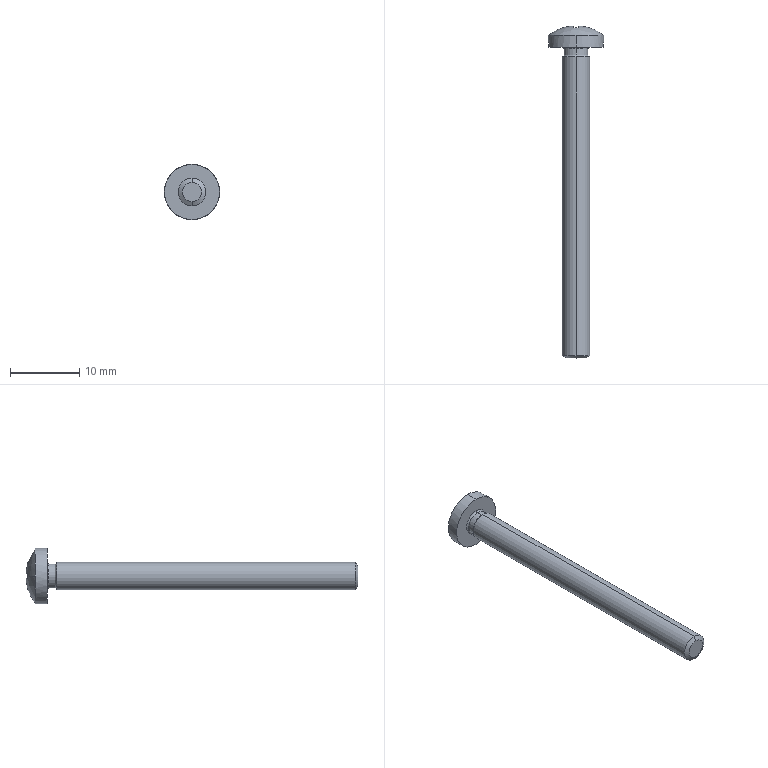Component | SolidWorks | GB_T818-2000PhillipsPanHeadScrewM4_45-1 | 1 solid | 28 faces | box 8 x 48.08 x 8 mm | volume 679 mm3 | plane 14 | cylinder 6 | cone 4 | torus 2 | sphere 2 | commonest cylinder face diameters 3.464 x2 8 x2 4 x2
build123d program:
from build123d import *


with BuildPart() as part:
    # Sketch2 → Base-Revolve (revolve)
    with BuildSketch(Plane.XY, mode=Mode.PRIVATE) as base_revolve_sk:
        with BuildLine():
            Line((0, 0), (48.1, 0))
            Line((48.1, 0), (48.1, 2))
            Line((48.1, 2), (4.5, 2))
            Line((4.5, 2), (4.232, 1.732))
            Line((4.232, 1.732), (3.318, 1.732))
            ThreePointArc((3.318, 1.732), (3.164, 1.796), (3.1, 1.95))
            Line((3.1, 1.95), (3.1, 4))
            Line((3.1, 4), (1.377, 4))
            ThreePointArc((1.377, 4), (0.3538, 2.115), (0, 0))
        make_face()
    revolve(base_revolve_sk.sketch.rotate(Axis((-1.332, 0, 0), (1, 0, 0)), 90), axis=Axis((-1.332, 0, 0), (1, 0, 0)))

    # Sketch3 → Cut-Revolve1 (revolve, cut)
    with BuildSketch(Plane.XY, mode=Mode.PRIVATE) as cut_revolve1_sk:
        Polygon((47.754, 2), (48.454, 2), (48.1, 1.394), align=None)
    revolve(cut_revolve1_sk.sketch.rotate(Axis((-0.2428, 0, 0), (1, 0, 0)), 90), axis=Axis((-0.2428, 0, 0), (1, 0, 0)), mode=Mode.SUBTRACT)

    # Sketch5 → Cut-Loft1 section 0
    with BuildSketch(Plane(origin=(0, 0, 0), x_dir=(0, 0, -1), z_dir=(1, 0, 0)), mode=Mode.PRIVATE) as cut_loft1_s0:
        with BuildLine():
            Line((0.35, 2.2), (-0.35, 2.2))
            Line((-0.35, 2.2), (-0.35, -2.2))
            Line((-0.35, -2.2), (0.35, -2.2))
            Line((0.35, -2.2), (0.35, 2.2))
        make_face()
    cut_loft1 = loft([Vertex(2.4, 0, 0), cut_loft1_s0.sketch], mode=Mode.SUBTRACT)

    # Mirror1: Cut-Loft1 across plane
    add(cut_loft1.mirror(Plane(origin=(0, 0, 0), x_dir=(0, 0.7071, 0.7071), z_dir=(0, -0.7071, 0.7071))), mode=Mode.SUBTRACT)


solid = part.part

# Placed as in the assembly
solid = solid.moved(Location((-141.534, 117.366, -146.507), (0, 0, -90)))
STEP:
#1=CARTESIAN_POINT('',(-5.572,2.727,-5.713));
#2=VERTEX_POINT('',#1);
#3=CARTESIAN_POINT('',(-5.572,2.727,-5.823));
#4=VERTEX_POINT('',#3);
#5=CARTESIAN_POINT('',(-5.572,2.727,-5.768));
#6=DIRECTION('',(0.,1.,0.));
#7=DIRECTION('',(0.,0.,1.));
#8=AXIS2_PLACEMENT_3D('',#5,#6,#7);
#9=CIRCLE('',#8,0.05487);
#10=EDGE_CURVE('',#2,#4,#9,.T.);
#11=ORIENTED_EDGE('',*,*,#10,.T.);
#12=CARTESIAN_POINT('',(-5.572,2.741,-5.847));
#13=VERTEX_POINT('',#12);
#14=CARTESIAN_POINT('',(-5.572,2.741,-5.847));
#15=DIRECTION('',(0.,0.4959,-0.8684));
#16=VECTOR('',#15,39.37);
#17=LINE('',#14,#16);
#18=EDGE_CURVE('',#4,#13,#17,.T.);
#19=ORIENTED_EDGE('',*,*,#18,.T.);
#20=CARTESIAN_POINT('',(-5.572,2.741,-5.689));
#21=VERTEX_POINT('',#20);
#22=CARTESIAN_POINT('',(-5.572,2.741,-5.768));
#23=DIRECTION('',(0.,1.,0.));
#24=DIRECTION('',(0.,0.,1.));
#25=AXIS2_PLACEMENT_3D('',#22,#23,#24);
#26=CIRCLE('',#25,0.07874);
#27=EDGE_CURVE('',#21,#13,#26,.T.);
#28=ORIENTED_EDGE('',*,*,#27,.F.);
#29=CARTESIAN_POINT('',(-5.572,2.741,-5.689));
#30=DIRECTION('',(0.,0.4959,0.8684));
#31=VECTOR('',#30,39.37);
#32=LINE('',#29,#31);
#33=EDGE_CURVE('',#2,#21,#32,.T.);
#34=ORIENTED_EDGE('',*,*,#33,.F.);
#35=EDGE_LOOP('',(#11,#19,#28,#34));
#36=FACE_OUTER_BOUND('',#35,.T.);
#37=CARTESIAN_POINT('',(-5.572,2.741,-5.768));
#38=DIRECTION('',(0.,1.,0.));
#39=DIRECTION('',(0.,0.,1.));
#40=AXIS2_PLACEMENT_3D('',#37,#38,#39);
#41=CONICAL_SURFACE('',#40,0.07874,1.052);
#42=ADVANCED_FACE('',(#36),#41,.T.);
#43=CARTESIAN_POINT('',(-5.572,4.454,-5.7));
#44=VERTEX_POINT('',#43);
#45=CARTESIAN_POINT('',(-5.572,4.454,-5.836));
#46=VERTEX_POINT('',#45);
#47=CARTESIAN_POINT('',(-5.572,4.454,-5.768));
#48=DIRECTION('',(0.,1.,0.));
#49=DIRECTION('',(0.,0.,1.));
#50=AXIS2_PLACEMENT_3D('',#47,#48,#49);
#51=CIRCLE('',#50,0.06819);
#52=EDGE_CURVE('',#44,#46,#51,.T.);
#53=ORIENTED_EDGE('',*,*,#52,.F.);
#54=CARTESIAN_POINT('',(-5.572,4.444,-5.689));
#55=VERTEX_POINT('',#54);
#56=CARTESIAN_POINT('',(-5.572,4.444,-5.689));
#57=DIRECTION('',(0.,-0.7071,0.7071));
#58=VECTOR('',#57,39.37);
#59=LINE('',#56,#58);
#60=EDGE_CURVE('',#44,#55,#59,.T.);
#61=ORIENTED_EDGE('',*,*,#60,.T.);
#62=CARTESIAN_POINT('',(-5.572,4.444,-5.847));
#63=VERTEX_POINT('',#62);
#64=CARTESIAN_POINT('',(-5.572,4.444,-5.768));
#65=DIRECTION('',(0.,1.,0.));
#66=DIRECTION('',(0.,0.,1.));
#67=AXIS2_PLACEMENT_3D('',#64,#65,#66);
#68=CIRCLE('',#67,0.07874);
#69=EDGE_CURVE('',#55,#63,#68,.T.);
#70=ORIENTED_EDGE('',*,*,#69,.T.);
#71=CARTESIAN_POINT('',(-5.572,4.444,-5.847));
#72=DIRECTION('',(0.,-0.7071,-0.7071));
#73=VECTOR('',#72,39.37);
#74=LINE('',#71,#73);
#75=EDGE_CURVE('',#46,#63,#74,.T.);
#76=ORIENTED_EDGE('',*,*,#75,.F.);
#77=EDGE_LOOP('',(#53,#61,#70,#76));
#78=FACE_OUTER_BOUND('',#77,.T.);
#79=CARTESIAN_POINT('',(-5.572,4.444,-5.768));
#80=DIRECTION('',(0.,-1.,0.));
#81=DIRECTION('',(0.,0.,-1.));
#82=AXIS2_PLACEMENT_3D('',#79,#80,#81);
#83=CONICAL_SURFACE('',#82,0.07874,0.7854);
#84=ADVANCED_FACE('',(#78),#83,.T.);
#85=ORIENTED_EDGE('',*,*,#52,.T.);
#86=CARTESIAN_POINT('',(-5.572,4.49,-5.836));
#87=VERTEX_POINT('',#86);
#88=CARTESIAN_POINT('',(-5.572,4.673,-5.836));
#89=DIRECTION('',(0.,1.,0.));
#90=VECTOR('',#89,39.37);
#91=LINE('',#88,#90);
#92=EDGE_CURVE('',#46,#87,#91,.T.);
#93=ORIENTED_EDGE('',*,*,#92,.T.);
#94=CARTESIAN_POINT('',(-5.572,4.49,-5.7));
#95=VERTEX_POINT('',#94);
#96=CARTESIAN_POINT('',(-5.572,4.49,-5.768));
#97=DIRECTION('',(0.,1.,0.));
#98=DIRECTION('',(0.,0.,1.));
#99=AXIS2_PLACEMENT_3D('',#96,#97,#98);
#100=CIRCLE('',#99,0.06819);
#101=EDGE_CURVE('',#95,#87,#100,.T.);
#102=ORIENTED_EDGE('',*,*,#101,.F.);
#103=CARTESIAN_POINT('',(-5.572,4.673,-5.7));
#104=DIRECTION('',(0.,1.,0.));
#105=VECTOR('',#104,39.37);
#106=LINE('',#103,#105);
#107=EDGE_CURVE('',#44,#95,#106,.T.);
#108=ORIENTED_EDGE('',*,*,#107,.F.);
#109=EDGE_LOOP('',(#85,#93,#102,#108));
#110=FACE_OUTER_BOUND('',#109,.T.);
#111=CARTESIAN_POINT('',(-5.572,4.673,-5.768));
#112=DIRECTION('',(0.,1.,0.));
#113=DIRECTION('',(0.,0.,1.));
#114=AXIS2_PLACEMENT_3D('',#111,#112,#113);
#115=CYLINDRICAL_SURFACE('',#114,0.06819);
#116=ADVANCED_FACE('',(#110),#115,.T.);
#117=CARTESIAN_POINT('',(-5.572,4.499,-5.845));
#118=VERTEX_POINT('',#117);
#119=CARTESIAN_POINT('',(-5.572,4.499,-5.691));
#120=VERTEX_POINT('',#119);
#121=CARTESIAN_POINT('',(-5.572,4.499,-5.768));
#122=DIRECTION('',(0.,1.,0.));
#123=DIRECTION('',(0.,0.,1.));
#124=AXIS2_PLACEMENT_3D('',#121,#122,#123);
#125=CIRCLE('',#124,0.07677);
#126=EDGE_CURVE('',#118,#120,#125,.T.);
#127=ORIENTED_EDGE('',*,*,#126,.F.);
#128=CARTESIAN_POINT('',(-5.572,4.49,-5.845));
#129=DIRECTION('',(1.,0.,0.));
#130=DIRECTION('',(0.,0.,-1.));
#131=AXIS2_PLACEMENT_3D('',#128,#129,#130);
#132=CIRCLE('',#131,0.008583);
#133=EDGE_CURVE('',#118,#87,#132,.T.);
#134=ORIENTED_EDGE('',*,*,#133,.T.);
#135=CARTESIAN_POINT('',(-5.572,4.49,-5.768));
#136=DIRECTION('',(0.,1.,0.));
#137=DIRECTION('',(0.,0.,1.));
#138=AXIS2_PLACEMENT_3D('',#135,#136,#137);
#139=CIRCLE('',#138,0.06819);
#140=EDGE_CURVE('',#87,#95,#139,.T.);
#141=ORIENTED_EDGE('',*,*,#140,.T.);
#142=CARTESIAN_POINT('',(-5.572,4.49,-5.691));
#143=DIRECTION('',(-1.,0.,0.));
#144=DIRECTION('',(0.,0.,1.));
#145=AXIS2_PLACEMENT_3D('',#142,#143,#144);
#146=CIRCLE('',#145,0.008583);
#147=EDGE_CURVE('',#120,#95,#146,.T.);
#148=ORIENTED_EDGE('',*,*,#147,.F.);
#149=EDGE_LOOP('',(#127,#134,#141,#148));
#150=FACE_OUTER_BOUND('',#149,.T.);
#151=CARTESIAN_POINT('',(-5.572,4.49,-5.768));
#152=DIRECTION('',(0.,1.,0.));
#153=DIRECTION('',(0.,0.,1.));
#154=AXIS2_PLACEMENT_3D('',#151,#152,#153);
#155=TOROIDAL_SURFACE('',#154,0.07677,0.008583);
#156=ADVANCED_FACE('',(#150),#155,.F.);
#157=CARTESIAN_POINT('',(-5.572,4.499,-5.611));
#158=VERTEX_POINT('',#157);
#159=CARTESIAN_POINT('',(-5.572,4.499,-5.925));
#160=VERTEX_POINT('',#159);
#161=CARTESIAN_POINT('',(-5.572,4.499,-5.768));
#162=DIRECTION('',(0.,1.,0.));
#163=DIRECTION('',(0.,0.,1.));
#164=AXIS2_PLACEMENT_3D('',#161,#162,#163);
#165=CIRCLE('',#164,0.1575);
#166=EDGE_CURVE('',#158,#160,#165,.T.);
#167=ORIENTED_EDGE('',*,*,#166,.T.);
#168=CARTESIAN_POINT('',(-5.572,4.567,-5.925));
#169=VERTEX_POINT('',#168);
#170=CARTESIAN_POINT('',(-5.572,4.673,-5.925));
#171=DIRECTION('',(0.,1.,0.));
#172=VECTOR('',#171,39.37);
#173=LINE('',#170,#172);
#174=EDGE_CURVE('',#160,#169,#173,.T.);
#175=ORIENTED_EDGE('',*,*,#174,.T.);
#176=CARTESIAN_POINT('',(-5.415,4.567,-5.768));
#177=VERTEX_POINT('',#176);
#178=CARTESIAN_POINT('',(-5.572,4.567,-5.768));
#179=DIRECTION('',(0.,1.,0.));
#180=DIRECTION('',(0.,0.,1.));
#181=AXIS2_PLACEMENT_3D('',#178,#179,#180);
#182=CIRCLE('',#181,0.1575);
#183=EDGE_CURVE('',#177,#169,#182,.T.);
#184=ORIENTED_EDGE('',*,*,#183,.F.);
#185=CARTESIAN_POINT('',(-5.572,4.567,-5.611));
#186=VERTEX_POINT('',#185);
#187=CARTESIAN_POINT('',(-5.572,4.567,-5.768));
#188=DIRECTION('',(0.,1.,0.));
#189=DIRECTION('',(0.,0.,1.));
#190=AXIS2_PLACEMENT_3D('',#187,#188,#189);
#191=CIRCLE('',#190,0.1575);
#192=EDGE_CURVE('',#186,#177,#191,.T.);
#193=ORIENTED_EDGE('',*,*,#192,.F.);
#194=CARTESIAN_POINT('',(-5.572,4.673,-5.611));
#195=DIRECTION('',(0.,1.,0.));
#196=VECTOR('',#195,39.37);
#197=LINE('',#194,#196);
#198=EDGE_CURVE('',#158,#186,#197,.T.);
#199=ORIENTED_EDGE('',*,*,#198,.F.);
#200=EDGE_LOOP('',(#167,#175,#184,#193,#199));
#201=FACE_OUTER_BOUND('',#200,.T.);
#202=CARTESIAN_POINT('',(-5.572,4.673,-5.768));
#203=DIRECTION('',(0.,1.,0.));
#204=DIRECTION('',(0.,0.,1.));
#205=AXIS2_PLACEMENT_3D('',#202,#203,#204);
#206=CYLINDRICAL_SURFACE('',#205,0.1575);
#207=ADVANCED_FACE('',(#201),#206,.T.);
#208=ORIENTED_EDGE('',*,*,#183,.T.);
#209=CARTESIAN_POINT('',(-5.73,4.567,-5.768));
#210=VERTEX_POINT('',#209);
#211=CARTESIAN_POINT('',(-5.572,4.567,-5.768));
#212=DIRECTION('',(0.,1.,0.));
#213=DIRECTION('',(0.,0.,1.));
#214=AXIS2_PLACEMENT_3D('',#211,#212,#213);
#215=CIRCLE('',#214,0.1575);
#216=EDGE_CURVE('',#169,#210,#215,.T.);
#217=ORIENTED_EDGE('',*,*,#216,.T.);
#218=CARTESIAN_POINT('',(-5.648,4.609,-5.768));
#219=VERTEX_POINT('',#218);
#220=CARTESIAN_POINT('',(-5.572,4.365,-5.768));
#221=DIRECTION('',(0.,0.,-1.));
#222=DIRECTION('',(-1.,0.,0.));
#223=AXIS2_PLACEMENT_3D('',#220,#221,#222);
#224=CIRCLE('',#223,0.2559);
#225=EDGE_CURVE('',#210,#219,#224,.T.);
#226=ORIENTED_EDGE('',*,*,#225,.T.);
#227=CARTESIAN_POINT('',(-5.648,4.609,-5.78));
#228=VERTEX_POINT('',#227);
#229=CARTESIAN_POINT('',(-5.492,4.439,-5.768));
#230=DIRECTION('',(-0.7372,-0.6757,0.));
#231=DIRECTION('',(0.6757,-0.7372,0.));
#232=AXIS2_PLACEMENT_3D('',#229,#230,#231);
#233=CIRCLE('',#232,0.2315);
#234=EDGE_CURVE('',#219,#228,#233,.T.);
#235=ORIENTED_EDGE('',*,*,#234,.T.);
#236=CARTESIAN_POINT('',(-5.586,4.62,-5.782));
#237=VERTEX_POINT('',#236);
#238=CARTESIAN_POINT('',(-5.572,4.368,-5.745));
#239=DIRECTION('',(0.,-0.1443,-0.9895));
#240=DIRECTION('',(0.,0.9895,-0.1443));
#241=AXIS2_PLACEMENT_3D('',#238,#239,#240);
#242=CIRCLE('',#241,0.2548);
#243=EDGE_CURVE('',#228,#237,#242,.T.);
#244=ORIENTED_EDGE('',*,*,#243,.T.);
#245=CARTESIAN_POINT('',(-5.584,4.609,-5.844));
#246=VERTEX_POINT('',#245);
#247=CARTESIAN_POINT('',(-5.549,4.368,-5.768));
#248=DIRECTION('',(-0.9895,-0.1443,-0.));
#249=DIRECTION('',(0.1443,-0.9895,0.));
#250=AXIS2_PLACEMENT_3D('',#247,#248,#249);
#251=CIRCLE('',#250,0.2548);
#252=EDGE_CURVE('',#237,#246,#251,.T.);
#253=ORIENTED_EDGE('',*,*,#252,.T.);
#254=CARTESIAN_POINT('',(-5.56,4.609,-5.844));
#255=VERTEX_POINT('',#254);
#256=CARTESIAN_POINT('',(-5.572,4.439,-5.688));
#257=DIRECTION('',(0.,-0.6757,-0.7372));
#258=DIRECTION('',(0.,0.7372,-0.6757));
#259=AXIS2_PLACEMENT_3D('',#256,#257,#258);
#260=CIRCLE('',#259,0.2315);
#261=EDGE_CURVE('',#246,#255,#260,.T.);
#262=ORIENTED_EDGE('',*,*,#261,.T.);
#263=CARTESIAN_POINT('',(-5.559,4.62,-5.782));
#264=VERTEX_POINT('',#263);
#265=CARTESIAN_POINT('',(-5.595,4.368,-5.768));
#266=DIRECTION('',(0.9895,-0.1443,0.));
#267=DIRECTION('',(0.1443,0.9895,0.));
#268=AXIS2_PLACEMENT_3D('',#265,#266,#267);
#269=CIRCLE('',#268,0.2548);
#270=EDGE_CURVE('',#255,#264,#269,.T.);
#271=ORIENTED_EDGE('',*,*,#270,.T.);
#272=CARTESIAN_POINT('',(-5.496,4.609,-5.78));
#273=VERTEX_POINT('',#272);
#274=CARTESIAN_POINT('',(-5.572,4.368,-5.745));
#275=DIRECTION('',(0.,-0.1443,-0.9895));
#276=DIRECTION('',(0.,0.9895,-0.1443));
#277=AXIS2_PLACEMENT_3D('',#274,#275,#276);
#278=CIRCLE('',#277,0.2548);
#279=EDGE_CURVE('',#264,#273,#278,.T.);
#280=ORIENTED_EDGE('',*,*,#279,.T.);
#281=CARTESIAN_POINT('',(-5.496,4.609,-5.768));
#282=VERTEX_POINT('',#281);
#283=CARTESIAN_POINT('',(-5.653,4.439,-5.768));
#284=DIRECTION('',(0.7372,-0.6757,0.));
#285=DIRECTION('',(0.6757,0.7372,0.));
#286=AXIS2_PLACEMENT_3D('',#283,#284,#285);
#287=CIRCLE('',#286,0.2315);
#288=EDGE_CURVE('',#273,#282,#287,.T.);
#289=ORIENTED_EDGE('',*,*,#288,.T.);
#290=CARTESIAN_POINT('',(-5.572,4.365,-5.768));
#291=DIRECTION('',(0.,0.,1.));
#292=DIRECTION('',(1.,0.,0.));
#293=AXIS2_PLACEMENT_3D('',#290,#291,#292);
#294=CIRCLE('',#293,0.2559);
#295=EDGE_CURVE('',#177,#282,#294,.T.);
#296=ORIENTED_EDGE('',*,*,#295,.F.);
#297=EDGE_LOOP('',(#208,#217,#226,#235,#244,#253,#262,#271,#280,#289,#296));
#298=FACE_OUTER_BOUND('',#297,.T.);
#299=CARTESIAN_POINT('',(-5.572,4.365,-5.768));
#300=DIRECTION('',(0.,0.,-1.));
#301=DIRECTION('',(1.,0.,0.));
#302=AXIS2_PLACEMENT_3D('',#299,#300,#301);
#303=SPHERICAL_SURFACE('',#302,0.2559);
#304=ADVANCED_FACE('',(#298),#303,.T.);
#305=ORIENTED_EDGE('',*,*,#27,.T.);
#306=CARTESIAN_POINT('',(-5.572,4.673,-5.847));
#307=DIRECTION('',(0.,1.,0.));
#308=VECTOR('',#307,39.37);
#309=LINE('',#306,#308);
#310=EDGE_CURVE('',#13,#63,#309,.T.);
#311=ORIENTED_EDGE('',*,*,#310,.T.);
#312=ORIENTED_EDGE('',*,*,#69,.F.);
#313=CARTESIAN_POINT('',(-5.572,4.673,-5.689));
#314=DIRECTION('',(0.,1.,0.));
#315=VECTOR('',#314,39.37);
#316=LINE('',#313,#315);
#317=EDGE_CURVE('',#21,#55,#316,.T.);
#318=ORIENTED_EDGE('',*,*,#317,.F.);
#319=EDGE_LOOP('',(#305,#311,#312,#318));
#320=FACE_OUTER_BOUND('',#319,.T.);
#321=CARTESIAN_POINT('',(-5.572,4.673,-5.768));
#322=DIRECTION('',(0.,1.,0.));
#323=DIRECTION('',(0.,0.,1.));
#324=AXIS2_PLACEMENT_3D('',#321,#322,#323);
#325=CYLINDRICAL_SURFACE('',#324,0.07874);
#326=ADVANCED_FACE('',(#320),#325,.T.);
#327=CARTESIAN_POINT('',(-5.572,4.526,-5.768));
#328=VERTEX_POINT('',#327);
#329=CARTESIAN_POINT('',(-5.572,4.526,-5.768));
#330=DIRECTION('',(-0.6719,0.7329,-0.1069));
#331=VECTOR('',#330,39.37);
#332=LINE('',#329,#331);
#333=EDGE_CURVE('',#328,#228,#332,.T.);
#334=ORIENTED_EDGE('',*,*,#333,.F.);
#335=CARTESIAN_POINT('',(-5.572,4.526,-5.768));
#336=DIRECTION('',(-0.1428,0.9794,-0.1428));
#337=VECTOR('',#336,39.37);
#338=LINE('',#335,#337);
#339=EDGE_CURVE('',#328,#237,#338,.T.);
#340=ORIENTED_EDGE('',*,*,#339,.T.);
#341=ORIENTED_EDGE('',*,*,#243,.F.);
#342=EDGE_LOOP('',(#334,#340,#341));
#343=FACE_OUTER_BOUND('',#342,.T.);
#344=CARTESIAN_POINT('',(-5.572,4.526,-5.768));
#345=DIRECTION('',(0.,-0.1443,-0.9895));
#346=DIRECTION('',(0.,0.9895,-0.1443));
#347=AXIS2_PLACEMENT_3D('',#344,#345,#346);
#348=PLANE('',#347);
#349=ADVANCED_FACE('',(#343),#348,.F.);
#350=CARTESIAN_POINT('',(-5.586,4.62,-5.754));
#351=VERTEX_POINT('',#350);
#352=CARTESIAN_POINT('',(-5.648,4.609,-5.756));
#353=VERTEX_POINT('',#352);
#354=CARTESIAN_POINT('',(-5.572,4.368,-5.791));
#355=DIRECTION('',(0.,-0.1443,0.9895));
#356=DIRECTION('',(0.,-0.9895,-0.1443));
#357=AXIS2_PLACEMENT_3D('',#354,#355,#356);
#358=CIRCLE('',#357,0.2548);
#359=EDGE_CURVE('',#351,#353,#358,.T.);
#360=ORIENTED_EDGE('',*,*,#359,.F.);
#361=CARTESIAN_POINT('',(-5.572,4.526,-5.768));
#362=DIRECTION('',(0.1428,-0.9794,-0.1428));
#363=VECTOR('',#362,39.37);
#364=LINE('',#361,#363);
#365=EDGE_CURVE('',#351,#328,#364,.T.);
#366=ORIENTED_EDGE('',*,*,#365,.T.);
#367=CARTESIAN_POINT('',(-5.572,4.526,-5.768));
#368=DIRECTION('',(-0.6719,0.7329,0.1069));
#369=VECTOR('',#368,39.37);
#370=LINE('',#367,#369);
#371=EDGE_CURVE('',#328,#353,#370,.T.);
#372=ORIENTED_EDGE('',*,*,#371,.T.);
#373=EDGE_LOOP('',(#360,#366,#372));
#374=FACE_OUTER_BOUND('',#373,.T.);
#375=CARTESIAN_POINT('',(-5.572,4.526,-5.768));
#376=DIRECTION('',(0.,-0.1443,0.9895));
#377=DIRECTION('',(0.,-0.9895,-0.1443));
#378=AXIS2_PLACEMENT_3D('',#375,#376,#377);
#379=PLANE('',#378);
#380=ADVANCED_FACE('',(#374),#379,.F.);
#381=ORIENTED_EDGE('',*,*,#310,.F.);
#382=CARTESIAN_POINT('',(-5.572,2.741,-5.768));
#383=DIRECTION('',(0.,1.,0.));
#384=DIRECTION('',(0.,0.,1.));
#385=AXIS2_PLACEMENT_3D('',#382,#383,#384);
#386=CIRCLE('',#385,0.07874);
#387=EDGE_CURVE('',#13,#21,#386,.T.);
#388=ORIENTED_EDGE('',*,*,#387,.T.);
#389=ORIENTED_EDGE('',*,*,#317,.T.);
#390=CARTESIAN_POINT('',(-5.572,4.444,-5.768));
#391=DIRECTION('',(0.,1.,0.));
#392=DIRECTION('',(0.,0.,1.));
#393=AXIS2_PLACEMENT_3D('',#390,#391,#392);
#394=CIRCLE('',#393,0.07874);
#395=EDGE_CURVE('',#63,#55,#394,.T.);
#396=ORIENTED_EDGE('',*,*,#395,.F.);
#397=EDGE_LOOP('',(#381,#388,#389,#396));
#398=FACE_OUTER_BOUND('',#397,.T.);
#399=CARTESIAN_POINT('',(-5.572,4.673,-5.768));
#400=DIRECTION('',(0.,1.,0.));
#401=DIRECTION('',(0.,0.,1.));
#402=AXIS2_PLACEMENT_3D('',#399,#400,#401);
#403=CYLINDRICAL_SURFACE('',#402,0.07874);
#404=ADVANCED_FACE('',(#398),#403,.T.);
#405=ORIENTED_EDGE('',*,*,#225,.F.);
#406=CARTESIAN_POINT('',(-5.572,4.567,-5.768));
#407=DIRECTION('',(0.,1.,0.));
#408=DIRECTION('',(0.,0.,1.));
#409=AXIS2_PLACEMENT_3D('',#406,#407,#408);
#410=CIRCLE('',#409,0.1575);
#411=EDGE_CURVE('',#210,#186,#410,.T.);
#412=ORIENTED_EDGE('',*,*,#411,.T.);
#413=ORIENTED_EDGE('',*,*,#192,.T.);
#414=ORIENTED_EDGE('',*,*,#295,.T.);
#415=CARTESIAN_POINT('',(-5.496,4.609,-5.756));
#416=VERTEX_POINT('',#415);
#417=CARTESIAN_POINT('',(-5.653,4.439,-5.768));
#418=DIRECTION('',(0.7372,-0.6757,0.));
#419=DIRECTION('',(0.6757,0.7372,0.));
#420=AXIS2_PLACEMENT_3D('',#417,#418,#419);
#421=CIRCLE('',#420,0.2315);
#422=EDGE_CURVE('',#282,#416,#421,.T.);
#423=ORIENTED_EDGE('',*,*,#422,.T.);
#424=CARTESIAN_POINT('',(-5.559,4.62,-5.754));
#425=VERTEX_POINT('',#424);
#426=CARTESIAN_POINT('',(-5.572,4.368,-5.791));
#427=DIRECTION('',(0.,-0.1443,0.9895));
#428=DIRECTION('',(0.,-0.9895,-0.1443));
#429=AXIS2_PLACEMENT_3D('',#426,#427,#428);
#430=CIRCLE('',#429,0.2548);
#431=EDGE_CURVE('',#416,#425,#430,.T.);
#432=ORIENTED_EDGE('',*,*,#431,.T.);
#433=CARTESIAN_POINT('',(-5.56,4.609,-5.692));
#434=VERTEX_POINT('',#433);
#435=CARTESIAN_POINT('',(-5.595,4.368,-5.768));
#436=DIRECTION('',(0.9895,-0.1443,0.));
#437=DIRECTION('',(0.1443,0.9895,0.));
#438=AXIS2_PLACEMENT_3D('',#435,#436,#437);
#439=CIRCLE('',#438,0.2548);
#440=EDGE_CURVE('',#425,#434,#439,.T.);
#441=ORIENTED_EDGE('',*,*,#440,.T.);
#442=CARTESIAN_POINT('',(-5.584,4.609,-5.692));
#443=VERTEX_POINT('',#442);
#444=CARTESIAN_POINT('',(-5.572,4.439,-5.848));
#445=DIRECTION('',(-0.,-0.6757,0.7372));
#446=DIRECTION('',(0.,-0.7372,-0.6757));
#447=AXIS2_PLACEMENT_3D('',#444,#445,#446);
#448=CIRCLE('',#447,0.2315);
#449=EDGE_CURVE('',#434,#443,#448,.T.);
#450=ORIENTED_EDGE('',*,*,#449,.T.);
#451=CARTESIAN_POINT('',(-5.549,4.368,-5.768));
#452=DIRECTION('',(-0.9895,-0.1443,-0.));
#453=DIRECTION('',(0.1443,-0.9895,0.));
#454=AXIS2_PLACEMENT_3D('',#451,#452,#453);
#455=CIRCLE('',#454,0.2548);
#456=EDGE_CURVE('',#443,#351,#455,.T.);
#457=ORIENTED_EDGE('',*,*,#456,.T.);
#458=ORIENTED_EDGE('',*,*,#359,.T.);
#459=CARTESIAN_POINT('',(-5.492,4.439,-5.768));
#460=DIRECTION('',(-0.7372,-0.6757,0.));
#461=DIRECTION('',(0.6757,-0.7372,0.));
#462=AXIS2_PLACEMENT_3D('',#459,#460,#461);
#463=CIRCLE('',#462,0.2315);
#464=EDGE_CURVE('',#353,#219,#463,.T.);
#465=ORIENTED_EDGE('',*,*,#464,.T.);
#466=EDGE_LOOP('',(#405,#412,#413,#414,#423,#432,#441,#450,#457,#458,#465));
#467=FACE_OUTER_BOUND('',#466,.T.);
#468=CARTESIAN_POINT('',(-5.572,4.365,-5.768));
#469=DIRECTION('',(0.,0.,-1.));
#470=DIRECTION('',(1.,0.,0.));
#471=AXIS2_PLACEMENT_3D('',#468,#469,#470);
#472=SPHERICAL_SURFACE('',#471,0.2559);
#473=ADVANCED_FACE('',(#467),#472,.T.);
#474=ORIENTED_EDGE('',*,*,#174,.F.);
#475=CARTESIAN_POINT('',(-5.572,4.499,-5.768));
#476=DIRECTION('',(0.,1.,0.));
#477=DIRECTION('',(0.,0.,1.));
#478=AXIS2_PLACEMENT_3D('',#475,#476,#477);
#479=CIRCLE('',#478,0.1575);
#480=EDGE_CURVE('',#160,#158,#479,.T.);
#481=ORIENTED_EDGE('',*,*,#480,.T.);
#482=ORIENTED_EDGE('',*,*,#198,.T.);
#483=ORIENTED_EDGE('',*,*,#411,.F.);
#484=ORIENTED_EDGE('',*,*,#216,.F.);
#485=EDGE_LOOP('',(#474,#481,#482,#483,#484));
#486=FACE_OUTER_BOUND('',#485,.T.);
#487=CARTESIAN_POINT('',(-5.572,4.673,-5.768));
#488=DIRECTION('',(0.,1.,0.));
#489=DIRECTION('',(0.,0.,1.));
#490=AXIS2_PLACEMENT_3D('',#487,#488,#489);
#491=CYLINDRICAL_SURFACE('',#490,0.1575);
#492=ADVANCED_FACE('',(#486),#491,.T.);
#493=ORIENTED_EDGE('',*,*,#166,.F.);
#494=ORIENTED_EDGE('',*,*,#480,.F.);
#495=EDGE_LOOP('',(#493,#494));
#496=FACE_OUTER_BOUND('',#495,.T.);
#497=CARTESIAN_POINT('',(-5.572,4.499,-5.768));
#498=DIRECTION('',(0.,1.,0.));
#499=DIRECTION('',(0.,0.,1.));
#500=AXIS2_PLACEMENT_3D('',#497,#498,#499);
#501=CIRCLE('',#500,0.07677);
#502=EDGE_CURVE('',#120,#118,#501,.T.);
#503=ORIENTED_EDGE('',*,*,#502,.T.);
#504=ORIENTED_EDGE('',*,*,#126,.T.);
#505=EDGE_LOOP('',(#503,#504));
#506=FACE_BOUND('',#505,.T.);
#507=CARTESIAN_POINT('',(-5.495,4.499,-5.768));
#508=DIRECTION('',(0.,1.,0.));
#509=DIRECTION('',(0.,0.,1.));
#510=AXIS2_PLACEMENT_3D('',#507,#508,#509);
#511=PLANE('',#510);
#512=ADVANCED_FACE('',(#496,#506),#511,.F.);
#513=ORIENTED_EDGE('',*,*,#133,.F.);
#514=ORIENTED_EDGE('',*,*,#502,.F.);
#515=ORIENTED_EDGE('',*,*,#147,.T.);
#516=ORIENTED_EDGE('',*,*,#101,.T.);
#517=EDGE_LOOP('',(#513,#514,#515,#516));
#518=FACE_OUTER_BOUND('',#517,.T.);
#519=CARTESIAN_POINT('',(-5.572,4.49,-5.768));
#520=DIRECTION('',(0.,1.,0.));
#521=DIRECTION('',(0.,0.,1.));
#522=AXIS2_PLACEMENT_3D('',#519,#520,#521);
#523=TOROIDAL_SURFACE('',#522,0.07677,0.008583);
#524=ADVANCED_FACE('',(#518),#523,.F.);
#525=ORIENTED_EDGE('',*,*,#92,.F.);
#526=CARTESIAN_POINT('',(-5.572,4.454,-5.768));
#527=DIRECTION('',(0.,1.,0.));
#528=DIRECTION('',(0.,0.,1.));
#529=AXIS2_PLACEMENT_3D('',#526,#527,#528);
#530=CIRCLE('',#529,0.06819);
#531=EDGE_CURVE('',#46,#44,#530,.T.);
#532=ORIENTED_EDGE('',*,*,#531,.T.);
#533=ORIENTED_EDGE('',*,*,#107,.T.);
#534=ORIENTED_EDGE('',*,*,#140,.F.);
#535=EDGE_LOOP('',(#525,#532,#533,#534));
#536=FACE_OUTER_BOUND('',#535,.T.);
#537=CARTESIAN_POINT('',(-5.572,4.673,-5.768));
#538=DIRECTION('',(0.,1.,0.));
#539=DIRECTION('',(0.,0.,1.));
#540=AXIS2_PLACEMENT_3D('',#537,#538,#539);
#541=CYLINDRICAL_SURFACE('',#540,0.06819);
#542=ADVANCED_FACE('',(#536),#541,.T.);
#543=ORIENTED_EDGE('',*,*,#60,.F.);
#544=ORIENTED_EDGE('',*,*,#531,.F.);
#545=ORIENTED_EDGE('',*,*,#75,.T.);
#546=ORIENTED_EDGE('',*,*,#395,.T.);
#547=EDGE_LOOP('',(#543,#544,#545,#546));
#548=FACE_OUTER_BOUND('',#547,.T.);
#549=CARTESIAN_POINT('',(-5.572,4.444,-5.768));
#550=DIRECTION('',(0.,-1.,0.));
#551=DIRECTION('',(0.,0.,-1.));
#552=AXIS2_PLACEMENT_3D('',#549,#550,#551);
#553=CONICAL_SURFACE('',#552,0.07874,0.7854);
#554=ADVANCED_FACE('',(#548),#553,.T.);
#555=ORIENTED_EDGE('',*,*,#18,.F.);
#556=CARTESIAN_POINT('',(-5.572,2.727,-5.768));
#557=DIRECTION('',(0.,1.,0.));
#558=DIRECTION('',(0.,0.,1.));
#559=AXIS2_PLACEMENT_3D('',#556,#557,#558);
#560=CIRCLE('',#559,0.05487);
#561=EDGE_CURVE('',#4,#2,#560,.T.);
#562=ORIENTED_EDGE('',*,*,#561,.T.);
#563=ORIENTED_EDGE('',*,*,#33,.T.);
#564=ORIENTED_EDGE('',*,*,#387,.F.);
#565=EDGE_LOOP('',(#555,#562,#563,#564));
#566=FACE_OUTER_BOUND('',#565,.T.);
#567=CARTESIAN_POINT('',(-5.572,2.741,-5.768));
#568=DIRECTION('',(0.,1.,0.));
#569=DIRECTION('',(0.,0.,1.));
#570=AXIS2_PLACEMENT_3D('',#567,#568,#569);
#571=CONICAL_SURFACE('',#570,0.07874,1.052);
#572=ADVANCED_FACE('',(#566),#571,.T.);
#573=ORIENTED_EDGE('',*,*,#10,.F.);
#574=ORIENTED_EDGE('',*,*,#561,.F.);
#575=EDGE_LOOP('',(#573,#574));
#576=FACE_OUTER_BOUND('',#575,.T.);
#577=CARTESIAN_POINT('',(-5.572,2.727,-5.768));
#578=DIRECTION('',(0.,1.,0.));
#579=DIRECTION('',(0.,0.,1.));
#580=AXIS2_PLACEMENT_3D('',#577,#578,#579);
#581=PLANE('',#580);
#582=ADVANCED_FACE('',(#576),#581,.F.);
#583=ORIENTED_EDGE('',*,*,#279,.F.);
#584=CARTESIAN_POINT('',(-5.572,4.526,-5.768));
#585=DIRECTION('',(-0.1428,-0.9794,0.1428));
#586=VECTOR('',#585,39.37);
#587=LINE('',#584,#586);
#588=EDGE_CURVE('',#264,#328,#587,.T.);
#589=ORIENTED_EDGE('',*,*,#588,.T.);
#590=CARTESIAN_POINT('',(-5.572,4.526,-5.768));
#591=DIRECTION('',(0.6719,0.7329,-0.1069));
#592=VECTOR('',#591,39.37);
#593=LINE('',#590,#592);
#594=EDGE_CURVE('',#328,#273,#593,.T.);
#595=ORIENTED_EDGE('',*,*,#594,.T.);
#596=EDGE_LOOP('',(#583,#589,#595));
#597=FACE_OUTER_BOUND('',#596,.T.);
#598=CARTESIAN_POINT('',(-5.572,4.526,-5.768));
#599=DIRECTION('',(0.,-0.1443,-0.9895));
#600=DIRECTION('',(0.,0.9895,-0.1443));
#601=AXIS2_PLACEMENT_3D('',#598,#599,#600);
#602=PLANE('',#601);
#603=ADVANCED_FACE('',(#597),#602,.F.);
#604=ORIENTED_EDGE('',*,*,#594,.F.);
#605=CARTESIAN_POINT('',(-5.572,4.526,-5.768));
#606=DIRECTION('',(0.6719,0.7329,0.1069));
#607=VECTOR('',#606,39.37);
#608=LINE('',#605,#607);
#609=EDGE_CURVE('',#328,#416,#608,.T.);
#610=ORIENTED_EDGE('',*,*,#609,.T.);
#611=ORIENTED_EDGE('',*,*,#422,.F.);
#612=ORIENTED_EDGE('',*,*,#288,.F.);
#613=EDGE_LOOP('',(#604,#610,#611,#612));
#614=FACE_OUTER_BOUND('',#613,.T.);
#615=CARTESIAN_POINT('',(-5.486,4.621,-5.782));
#616=DIRECTION('',(0.7372,-0.6757,0.));
#617=DIRECTION('',(0.6757,0.7372,0.));
#618=AXIS2_PLACEMENT_3D('',#615,#616,#617);
#619=PLANE('',#618);
#620=ADVANCED_FACE('',(#614),#619,.F.);
#621=ORIENTED_EDGE('',*,*,#371,.F.);
#622=ORIENTED_EDGE('',*,*,#333,.T.);
#623=ORIENTED_EDGE('',*,*,#234,.F.);
#624=ORIENTED_EDGE('',*,*,#464,.F.);
#625=EDGE_LOOP('',(#621,#622,#623,#624));
#626=FACE_OUTER_BOUND('',#625,.T.);
#627=CARTESIAN_POINT('',(-5.659,4.621,-5.754));
#628=DIRECTION('',(-0.7372,-0.6757,0.));
#629=DIRECTION('',(0.6757,-0.7372,0.));
#630=AXIS2_PLACEMENT_3D('',#627,#628,#629);
#631=PLANE('',#630);
#632=ADVANCED_FACE('',(#626),#631,.F.);
#633=ORIENTED_EDGE('',*,*,#609,.F.);
#634=CARTESIAN_POINT('',(-5.572,4.526,-5.768));
#635=DIRECTION('',(0.1428,0.9794,0.1428));
#636=VECTOR('',#635,39.37);
#637=LINE('',#634,#636);
#638=EDGE_CURVE('',#328,#425,#637,.T.);
#639=ORIENTED_EDGE('',*,*,#638,.T.);
#640=ORIENTED_EDGE('',*,*,#431,.F.);
#641=EDGE_LOOP('',(#633,#639,#640));
#642=FACE_OUTER_BOUND('',#641,.T.);
#643=CARTESIAN_POINT('',(-5.572,4.526,-5.768));
#644=DIRECTION('',(0.,-0.1443,0.9895));
#645=DIRECTION('',(0.,-0.9895,-0.1443));
#646=AXIS2_PLACEMENT_3D('',#643,#644,#645);
#647=PLANE('',#646);
#648=ADVANCED_FACE('',(#642),#647,.F.);
#649=CARTESIAN_POINT('',(-5.572,4.526,-5.768));
#650=DIRECTION('',(-0.1069,0.7329,0.6719));
#651=VECTOR('',#650,39.37);
#652=LINE('',#649,#651);
#653=EDGE_CURVE('',#328,#443,#652,.T.);
#654=ORIENTED_EDGE('',*,*,#653,.F.);
#655=ORIENTED_EDGE('',*,*,#365,.F.);
#656=ORIENTED_EDGE('',*,*,#456,.F.);
#657=EDGE_LOOP('',(#654,#655,#656));
#658=FACE_OUTER_BOUND('',#657,.T.);
#659=CARTESIAN_POINT('',(-5.572,4.526,-5.768));
#660=DIRECTION('',(-0.9895,-0.1443,-0.));
#661=DIRECTION('',(-0.1443,0.9895,-0.));
#662=AXIS2_PLACEMENT_3D('',#659,#660,#661);
#663=PLANE('',#662);
#664=ADVANCED_FACE('',(#658),#663,.F.);
#665=ORIENTED_EDGE('',*,*,#638,.F.);
#666=CARTESIAN_POINT('',(-5.572,4.526,-5.768));
#667=DIRECTION('',(0.1069,0.7329,0.6719));
#668=VECTOR('',#667,39.37);
#669=LINE('',#666,#668);
#670=EDGE_CURVE('',#328,#434,#669,.T.);
#671=ORIENTED_EDGE('',*,*,#670,.T.);
#672=ORIENTED_EDGE('',*,*,#440,.F.);
#673=EDGE_LOOP('',(#665,#671,#672));
#674=FACE_OUTER_BOUND('',#673,.T.);
#675=CARTESIAN_POINT('',(-5.572,4.526,-5.768));
#676=DIRECTION('',(0.9895,-0.1443,0.));
#677=DIRECTION('',(-0.1443,-0.9895,-0.));
#678=AXIS2_PLACEMENT_3D('',#675,#676,#677);
#679=PLANE('',#678);
#680=ADVANCED_FACE('',(#674),#679,.F.);
#681=ORIENTED_EDGE('',*,*,#670,.F.);
#682=ORIENTED_EDGE('',*,*,#653,.T.);
#683=ORIENTED_EDGE('',*,*,#449,.F.);
#684=EDGE_LOOP('',(#681,#682,#683));
#685=FACE_OUTER_BOUND('',#684,.T.);
#686=CARTESIAN_POINT('',(-5.586,4.621,-5.681));
#687=DIRECTION('',(-0.,-0.6757,0.7372));
#688=DIRECTION('',(-0.,0.7372,0.6757));
#689=AXIS2_PLACEMENT_3D('',#686,#687,#688);
#690=PLANE('',#689);
#691=ADVANCED_FACE('',(#685),#690,.F.);
#692=ORIENTED_EDGE('',*,*,#339,.F.);
#693=CARTESIAN_POINT('',(-5.572,4.526,-5.768));
#694=DIRECTION('',(-0.1069,0.7329,-0.6719));
#695=VECTOR('',#694,39.37);
#696=LINE('',#693,#695);
#697=EDGE_CURVE('',#328,#246,#696,.T.);
#698=ORIENTED_EDGE('',*,*,#697,.T.);
#699=ORIENTED_EDGE('',*,*,#252,.F.);
#700=EDGE_LOOP('',(#692,#698,#699));
#701=FACE_OUTER_BOUND('',#700,.T.);
#702=CARTESIAN_POINT('',(-5.572,4.526,-5.768));
#703=DIRECTION('',(-0.9895,-0.1443,-0.));
#704=DIRECTION('',(-0.1443,0.9895,-0.));
#705=AXIS2_PLACEMENT_3D('',#702,#703,#704);
#706=PLANE('',#705);
#707=ADVANCED_FACE('',(#701),#706,.F.);
#708=ORIENTED_EDGE('',*,*,#697,.F.);
#709=CARTESIAN_POINT('',(-5.572,4.526,-5.768));
#710=DIRECTION('',(0.1069,0.7329,-0.6719));
#711=VECTOR('',#710,39.37);
#712=LINE('',#709,#711);
#713=EDGE_CURVE('',#328,#255,#712,.T.);
#714=ORIENTED_EDGE('',*,*,#713,.T.);
#715=ORIENTED_EDGE('',*,*,#261,.F.);
#716=EDGE_LOOP('',(#708,#714,#715));
#717=FACE_OUTER_BOUND('',#716,.T.);
#718=CARTESIAN_POINT('',(-5.558,4.621,-5.855));
#719=DIRECTION('',(0.,-0.6757,-0.7372));
#720=DIRECTION('',(-0.,-0.7372,0.6757));
#721=AXIS2_PLACEMENT_3D('',#718,#719,#720);
#722=PLANE('',#721);
#723=ADVANCED_FACE('',(#717),#722,.F.);
#724=ORIENTED_EDGE('',*,*,#713,.F.);
#725=ORIENTED_EDGE('',*,*,#588,.F.);
#726=ORIENTED_EDGE('',*,*,#270,.F.);
#727=EDGE_LOOP('',(#724,#725,#726));
#728=FACE_OUTER_BOUND('',#727,.T.);
#729=CARTESIAN_POINT('',(-5.572,4.526,-5.768));
#730=DIRECTION('',(0.9895,-0.1443,0.));
#731=DIRECTION('',(-0.1443,-0.9895,-0.));
#732=AXIS2_PLACEMENT_3D('',#729,#730,#731);
#733=PLANE('',#732);
#734=ADVANCED_FACE('',(#728),#733,.F.);
#735=CLOSED_SHELL('',(#42,#84,#116,#156,#207,#304,#326,#349,#380,#404,#473,#492,#512,#524,#542,#554,#572,#582,#603,#620,#632,#648,#664,#680,#691,#707,#723,#734));
#736=MANIFOLD_SOLID_BREP('',#735);
#737=CARTESIAN_POINT('',(0.,0.,0.));
#738=DIRECTION('',(0.,0.,1.));
#739=DIRECTION('',(1.,0.,0.));
#740=AXIS2_PLACEMENT_3D('',#737,#738,#739);
#741=(LENGTH_UNIT()NAMED_UNIT(*)SI_UNIT($,.METRE.));
#742=LENGTH_MEASURE_WITH_UNIT(LENGTH_MEASURE(0.0254),#741);
#743=DIMENSIONAL_EXPONENTS(1.,0.,0.,0.,0.,0.,0.);
#744=(CONVERSION_BASED_UNIT('',#742)LENGTH_UNIT()NAMED_UNIT(#743));
#745=UNCERTAINTY_MEASURE_WITH_UNIT(LENGTH_MEASURE(0.00001),#744,'','');
#746=(NAMED_UNIT(*)PLANE_ANGLE_UNIT()SI_UNIT($,.RADIAN.));
#747=(NAMED_UNIT(*)SI_UNIT($,.STERADIAN.)SOLID_ANGLE_UNIT());
#748=(GEOMETRIC_REPRESENTATION_CONTEXT(3)GLOBAL_UNCERTAINTY_ASSIGNED_CONTEXT((#745))GLOBAL_UNIT_ASSIGNED_CONTEXT((#744,#746,#747))REPRESENTATION_CONTEXT('',''));
#749=ADVANCED_BREP_SHAPE_REPRESENTATION('',(#736,#740),#748);
#750=COLOUR_RGB('',0.7922,0.8196,0.9333);
#751=FILL_AREA_STYLE_COLOUR('',#750);
#752=FILL_AREA_STYLE('',(#751));
#753=SURFACE_STYLE_FILL_AREA(#752);
#754=SURFACE_SIDE_STYLE('',(#753));
#755=SURFACE_STYLE_USAGE(.BOTH.,#754);
#756=PRESENTATION_STYLE_ASSIGNMENT((#755));
#757=STYLED_ITEM('',(#756),#736);
#758=(LENGTH_UNIT()NAMED_UNIT(*)SI_UNIT($,.METRE.));
#759=LENGTH_MEASURE_WITH_UNIT(LENGTH_MEASURE(0.0254),#758);
#760=DIMENSIONAL_EXPONENTS(1.,0.,0.,0.,0.,0.,0.);
#761=(CONVERSION_BASED_UNIT('',#759)LENGTH_UNIT()NAMED_UNIT(#760));
#762=UNCERTAINTY_MEASURE_WITH_UNIT(LENGTH_MEASURE(0.00001),#761,'','');
#763=(NAMED_UNIT(*)PLANE_ANGLE_UNIT()SI_UNIT($,.RADIAN.));
#764=(NAMED_UNIT(*)SI_UNIT($,.STERADIAN.)SOLID_ANGLE_UNIT());
#765=(GEOMETRIC_REPRESENTATION_CONTEXT(3)GLOBAL_UNCERTAINTY_ASSIGNED_CONTEXT((#762))GLOBAL_UNIT_ASSIGNED_CONTEXT((#761,#763,#764))REPRESENTATION_CONTEXT('',''));
#766=MECHANICAL_DESIGN_GEOMETRIC_PRESENTATION_REPRESENTATION('',(#757),#765);
#767=PRESENTATION_LAYER_ASSIGNMENT('','',(#757));